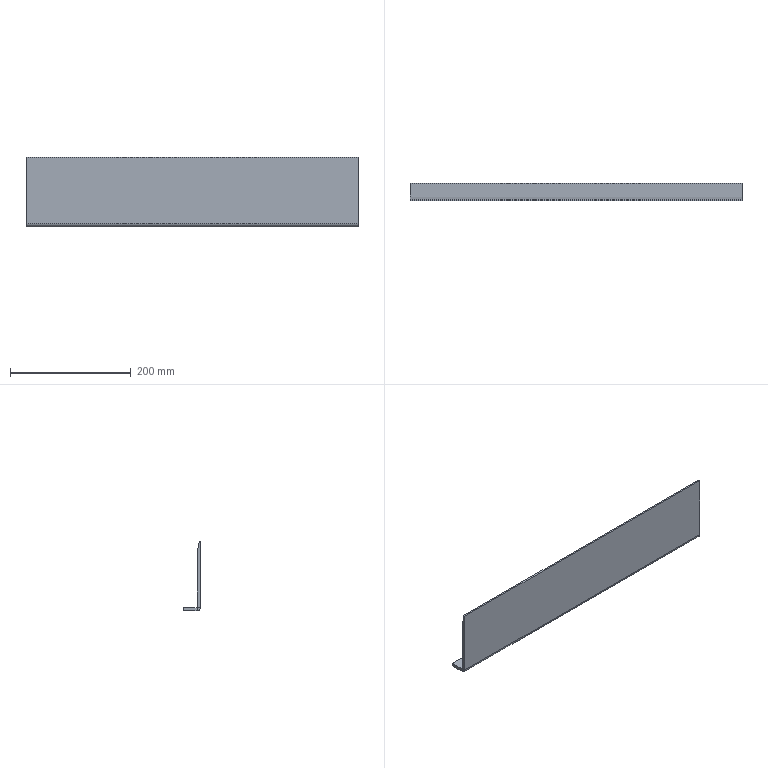Component | SolidWorks | PusherTray-1 | 1 solid | 15 faces | box 550 x 29 x 115.5 mm | volume 402219 mm3 | plane 13 | cylinder 2 | commonest cylinder face diameters 1 x1 12 x1
STEP:
#1=COLOUR_RGB('',0.7922,0.8196,0.9333);
#2=FILL_AREA_STYLE_COLOUR('',#1);
#3=FILL_AREA_STYLE('',(#2));
#4=SURFACE_STYLE_FILL_AREA(#3);
#5=SURFACE_SIDE_STYLE('',(#4));
#6=SURFACE_STYLE_USAGE(.BOTH.,#5);
#7=PRESENTATION_STYLE_ASSIGNMENT((#6));
#8=CARTESIAN_POINT('',(0.9843,24.724,0.8858));
#9=VERTEX_POINT('',#8);
#10=CARTESIAN_POINT('',(0.9843,24.508,0.8858));
#11=VERTEX_POINT('',#10);
#12=CARTESIAN_POINT('',(0.9843,24.724,0.8858));
#13=DIRECTION('',(0.,-1.,-0.));
#14=VECTOR('',#13,39.37);
#15=LINE('',#12,#14);
#16=EDGE_CURVE('',#9,#11,#15,.T.);
#17=ORIENTED_EDGE('',*,*,#16,.F.);
#18=CARTESIAN_POINT('',(0.9843,24.744,0.8661));
#19=VERTEX_POINT('',#18);
#20=CARTESIAN_POINT('',(0.9843,24.744,0.8858));
#21=DIRECTION('',(-1.,-0.,0.));
#22=DIRECTION('',(0.,0.,-1.));
#23=AXIS2_PLACEMENT_3D('',#20,#21,#22);
#24=CIRCLE('',#23,0.01969);
#25=EDGE_CURVE('',#19,#9,#24,.T.);
#26=ORIENTED_EDGE('',*,*,#25,.F.);
#27=CARTESIAN_POINT('',(0.9843,24.744,0.6496));
#28=VERTEX_POINT('',#27);
#29=CARTESIAN_POINT('',(0.9843,24.744,0.6496));
#30=DIRECTION('',(0.,-0.,1.));
#31=VECTOR('',#30,39.37);
#32=LINE('',#29,#31);
#33=EDGE_CURVE('',#28,#19,#32,.T.);
#34=ORIENTED_EDGE('',*,*,#33,.F.);
#35=CARTESIAN_POINT('',(0.9843,24.744,0.8858));
#36=DIRECTION('',(-1.,-0.,0.));
#37=DIRECTION('',(0.,0.,1.));
#38=AXIS2_PLACEMENT_3D('',#35,#36,#37);
#39=CIRCLE('',#38,0.2362);
#40=EDGE_CURVE('',#28,#11,#39,.T.);
#41=ORIENTED_EDGE('',*,*,#40,.T.);
#42=EDGE_LOOP('',(#17,#26,#34,#41));
#43=FACE_OUTER_BOUND('',#42,.T.);
#44=CARTESIAN_POINT('',(0.9843,24.724,0.8858));
#45=DIRECTION('',(-1.,-0.,0.));
#46=DIRECTION('',(0.,-0.,1.));
#47=AXIS2_PLACEMENT_3D('',#44,#45,#46);
#48=PLANE('',#47);
#49=ADVANCED_FACE('',(#43),#48,.T.);
#50=CARTESIAN_POINT('',(0.9843,24.606,5.197));
#51=VERTEX_POINT('',#50);
#52=CARTESIAN_POINT('',(0.9843,24.508,5.197));
#53=VERTEX_POINT('',#52);
#54=CARTESIAN_POINT('',(0.9843,24.724,5.197));
#55=DIRECTION('',(0.,-1.,-0.));
#56=VECTOR('',#55,39.37);
#57=LINE('',#54,#56);
#58=EDGE_CURVE('',#51,#53,#57,.T.);
#59=ORIENTED_EDGE('',*,*,#58,.F.);
#60=CARTESIAN_POINT('',(0.9843,24.724,4.527));
#61=VERTEX_POINT('',#60);
#62=CARTESIAN_POINT('',(0.9843,25.388,0.7632));
#63=DIRECTION('',(-0.,0.1736,-0.9848));
#64=VECTOR('',#63,39.37);
#65=LINE('',#62,#64);
#66=EDGE_CURVE('',#51,#61,#65,.T.);
#67=ORIENTED_EDGE('',*,*,#66,.T.);
#68=CARTESIAN_POINT('',(0.9843,24.724,0.8661));
#69=DIRECTION('',(0.,-0.,1.));
#70=VECTOR('',#69,39.37);
#71=LINE('',#68,#70);
#72=EDGE_CURVE('',#9,#61,#71,.T.);
#73=ORIENTED_EDGE('',*,*,#72,.F.);
#74=ORIENTED_EDGE('',*,*,#16,.T.);
#75=CARTESIAN_POINT('',(0.9843,24.508,0.8661));
#76=DIRECTION('',(0.,-0.,1.));
#77=VECTOR('',#76,39.37);
#78=LINE('',#75,#77);
#79=EDGE_CURVE('',#11,#53,#78,.T.);
#80=ORIENTED_EDGE('',*,*,#79,.T.);
#81=EDGE_LOOP('',(#59,#67,#73,#74,#80));
#82=FACE_OUTER_BOUND('',#81,.T.);
#83=CARTESIAN_POINT('',(0.9843,24.744,0.6496));
#84=DIRECTION('',(-1.,-0.,0.));
#85=DIRECTION('',(0.,-0.,1.));
#86=AXIS2_PLACEMENT_3D('',#83,#84,#85);
#87=PLANE('',#86);
#88=ADVANCED_FACE('',(#82),#87,.T.);
#89=CARTESIAN_POINT('',(22.638,24.744,0.8661));
#90=VERTEX_POINT('',#89);
#91=CARTESIAN_POINT('',(22.638,24.744,0.6496));
#92=VERTEX_POINT('',#91);
#93=CARTESIAN_POINT('',(22.638,24.744,0.8661));
#94=DIRECTION('',(-0.,0.,-1.));
#95=VECTOR('',#94,39.37);
#96=LINE('',#93,#95);
#97=EDGE_CURVE('',#90,#92,#96,.T.);
#98=ORIENTED_EDGE('',*,*,#97,.F.);
#99=CARTESIAN_POINT('',(22.638,24.724,0.8858));
#100=VERTEX_POINT('',#99);
#101=CARTESIAN_POINT('',(22.638,24.744,0.8858));
#102=DIRECTION('',(-1.,-0.,0.));
#103=DIRECTION('',(0.,0.,-1.));
#104=AXIS2_PLACEMENT_3D('',#101,#102,#103);
#105=CIRCLE('',#104,0.01969);
#106=EDGE_CURVE('',#90,#100,#105,.T.);
#107=ORIENTED_EDGE('',*,*,#106,.T.);
#108=CARTESIAN_POINT('',(22.638,24.508,0.8858));
#109=VERTEX_POINT('',#108);
#110=CARTESIAN_POINT('',(22.638,24.508,0.8858));
#111=DIRECTION('',(-0.,1.,0.));
#112=VECTOR('',#111,39.37);
#113=LINE('',#110,#112);
#114=EDGE_CURVE('',#109,#100,#113,.T.);
#115=ORIENTED_EDGE('',*,*,#114,.F.);
#116=CARTESIAN_POINT('',(22.638,24.744,0.8858));
#117=DIRECTION('',(-1.,-0.,0.));
#118=DIRECTION('',(0.,0.,1.));
#119=AXIS2_PLACEMENT_3D('',#116,#117,#118);
#120=CIRCLE('',#119,0.2362);
#121=EDGE_CURVE('',#92,#109,#120,.T.);
#122=ORIENTED_EDGE('',*,*,#121,.F.);
#123=EDGE_LOOP('',(#98,#107,#115,#122));
#124=FACE_OUTER_BOUND('',#123,.T.);
#125=CARTESIAN_POINT('',(22.638,24.744,0.8661));
#126=DIRECTION('',(1.,0.,-0.));
#127=DIRECTION('',(-0.,0.,-1.));
#128=AXIS2_PLACEMENT_3D('',#125,#126,#127);
#129=PLANE('',#128);
#130=ADVANCED_FACE('',(#124),#129,.T.);
#131=CARTESIAN_POINT('',(22.638,25.65,0.8661));
#132=VERTEX_POINT('',#131);
#133=CARTESIAN_POINT('',(22.638,24.724,0.8661));
#134=DIRECTION('',(0.,-1.,-0.));
#135=VECTOR('',#134,39.37);
#136=LINE('',#133,#135);
#137=EDGE_CURVE('',#132,#90,#136,.T.);
#138=ORIENTED_EDGE('',*,*,#137,.T.);
#139=ORIENTED_EDGE('',*,*,#97,.T.);
#140=CARTESIAN_POINT('',(22.638,25.65,0.6496));
#141=VERTEX_POINT('',#140);
#142=CARTESIAN_POINT('',(22.638,24.724,0.6496));
#143=DIRECTION('',(0.,-1.,-0.));
#144=VECTOR('',#143,39.37);
#145=LINE('',#142,#144);
#146=EDGE_CURVE('',#141,#92,#145,.T.);
#147=ORIENTED_EDGE('',*,*,#146,.F.);
#148=CARTESIAN_POINT('',(22.638,25.65,0.6496));
#149=DIRECTION('',(0.,-0.,1.));
#150=VECTOR('',#149,39.37);
#151=LINE('',#148,#150);
#152=EDGE_CURVE('',#141,#132,#151,.T.);
#153=ORIENTED_EDGE('',*,*,#152,.T.);
#154=EDGE_LOOP('',(#138,#139,#147,#153));
#155=FACE_OUTER_BOUND('',#154,.T.);
#156=CARTESIAN_POINT('',(22.638,24.508,0.8858));
#157=DIRECTION('',(1.,0.,-0.));
#158=DIRECTION('',(-0.,0.,-1.));
#159=AXIS2_PLACEMENT_3D('',#156,#157,#158);
#160=PLANE('',#159);
#161=ADVANCED_FACE('',(#155),#160,.T.);
#162=CARTESIAN_POINT('',(22.638,24.508,5.197));
#163=VERTEX_POINT('',#162);
#164=CARTESIAN_POINT('',(22.638,24.508,0.8661));
#165=DIRECTION('',(0.,-0.,1.));
#166=VECTOR('',#165,39.37);
#167=LINE('',#164,#166);
#168=EDGE_CURVE('',#109,#163,#167,.T.);
#169=ORIENTED_EDGE('',*,*,#168,.T.);
#170=CARTESIAN_POINT('',(0.9843,24.508,5.197));
#171=DIRECTION('',(1.,0.,-0.));
#172=VECTOR('',#171,39.37);
#173=LINE('',#170,#172);
#174=EDGE_CURVE('',#53,#163,#173,.T.);
#175=ORIENTED_EDGE('',*,*,#174,.F.);
#176=ORIENTED_EDGE('',*,*,#79,.F.);
#177=CARTESIAN_POINT('',(0.9843,24.508,0.8858));
#178=DIRECTION('',(1.,0.,-0.));
#179=VECTOR('',#178,39.37);
#180=LINE('',#177,#179);
#181=EDGE_CURVE('',#11,#109,#180,.T.);
#182=ORIENTED_EDGE('',*,*,#181,.T.);
#183=EDGE_LOOP('',(#169,#175,#176,#182));
#184=FACE_OUTER_BOUND('',#183,.T.);
#185=CARTESIAN_POINT('',(0.9843,24.508,0.8661));
#186=DIRECTION('',(-0.,1.,0.));
#187=DIRECTION('',(-1.,-0.,0.));
#188=AXIS2_PLACEMENT_3D('',#185,#186,#187);
#189=PLANE('',#188);
#190=ADVANCED_FACE('',(#184),#189,.F.);
#191=CARTESIAN_POINT('',(22.638,24.606,5.197));
#192=VERTEX_POINT('',#191);
#193=CARTESIAN_POINT('',(22.638,24.724,5.197));
#194=DIRECTION('',(0.,-1.,-0.));
#195=VECTOR('',#194,39.37);
#196=LINE('',#193,#195);
#197=EDGE_CURVE('',#192,#163,#196,.T.);
#198=ORIENTED_EDGE('',*,*,#197,.F.);
#199=CARTESIAN_POINT('',(0.9843,24.606,5.197));
#200=DIRECTION('',(-1.,-0.,0.));
#201=VECTOR('',#200,39.37);
#202=LINE('',#199,#201);
#203=EDGE_CURVE('',#192,#51,#202,.T.);
#204=ORIENTED_EDGE('',*,*,#203,.T.);
#205=ORIENTED_EDGE('',*,*,#58,.T.);
#206=ORIENTED_EDGE('',*,*,#174,.T.);
#207=EDGE_LOOP('',(#198,#204,#205,#206));
#208=FACE_OUTER_BOUND('',#207,.T.);
#209=CARTESIAN_POINT('',(0.9843,24.724,5.197));
#210=DIRECTION('',(0.,-0.,1.));
#211=DIRECTION('',(1.,0.,-0.));
#212=AXIS2_PLACEMENT_3D('',#209,#210,#211);
#213=PLANE('',#212);
#214=ADVANCED_FACE('',(#208),#213,.T.);
#215=ORIENTED_EDGE('',*,*,#72,.T.);
#216=CARTESIAN_POINT('',(22.638,24.724,4.527));
#217=VERTEX_POINT('',#216);
#218=CARTESIAN_POINT('',(0.9843,24.724,4.527));
#219=DIRECTION('',(1.,0.,-0.));
#220=VECTOR('',#219,39.37);
#221=LINE('',#218,#220);
#222=EDGE_CURVE('',#61,#217,#221,.T.);
#223=ORIENTED_EDGE('',*,*,#222,.T.);
#224=CARTESIAN_POINT('',(22.638,24.724,0.8661));
#225=DIRECTION('',(0.,-0.,1.));
#226=VECTOR('',#225,39.37);
#227=LINE('',#224,#226);
#228=EDGE_CURVE('',#100,#217,#227,.T.);
#229=ORIENTED_EDGE('',*,*,#228,.F.);
#230=CARTESIAN_POINT('',(0.9843,24.724,0.8858));
#231=DIRECTION('',(1.,0.,-0.));
#232=VECTOR('',#231,39.37);
#233=LINE('',#230,#232);
#234=EDGE_CURVE('',#9,#100,#233,.T.);
#235=ORIENTED_EDGE('',*,*,#234,.F.);
#236=EDGE_LOOP('',(#215,#223,#229,#235));
#237=FACE_OUTER_BOUND('',#236,.T.);
#238=CARTESIAN_POINT('',(0.9843,24.724,0.8661));
#239=DIRECTION('',(-0.,1.,0.));
#240=DIRECTION('',(-1.,-0.,0.));
#241=AXIS2_PLACEMENT_3D('',#238,#239,#240);
#242=PLANE('',#241);
#243=ADVANCED_FACE('',(#237),#242,.T.);
#244=ORIENTED_EDGE('',*,*,#106,.F.);
#245=CARTESIAN_POINT('',(0.9843,24.744,0.8661));
#246=DIRECTION('',(1.,0.,-0.));
#247=VECTOR('',#246,39.37);
#248=LINE('',#245,#247);
#249=EDGE_CURVE('',#19,#90,#248,.T.);
#250=ORIENTED_EDGE('',*,*,#249,.F.);
#251=ORIENTED_EDGE('',*,*,#25,.T.);
#252=ORIENTED_EDGE('',*,*,#234,.T.);
#253=EDGE_LOOP('',(#244,#250,#251,#252));
#254=FACE_OUTER_BOUND('',#253,.T.);
#255=CARTESIAN_POINT('',(0.9843,24.744,0.8858));
#256=DIRECTION('',(1.,0.,-0.));
#257=DIRECTION('',(0.,0.,-1.));
#258=AXIS2_PLACEMENT_3D('',#255,#256,#257);
#259=CYLINDRICAL_SURFACE('',#258,0.01969);
#260=ADVANCED_FACE('',(#254),#259,.F.);
#261=ORIENTED_EDGE('',*,*,#137,.F.);
#262=CARTESIAN_POINT('',(0.9843,25.65,0.8661));
#263=VERTEX_POINT('',#262);
#264=CARTESIAN_POINT('',(0.9843,25.65,0.8661));
#265=DIRECTION('',(1.,0.,-0.));
#266=VECTOR('',#265,39.37);
#267=LINE('',#264,#266);
#268=EDGE_CURVE('',#263,#132,#267,.T.);
#269=ORIENTED_EDGE('',*,*,#268,.F.);
#270=CARTESIAN_POINT('',(0.9843,24.724,0.8661));
#271=DIRECTION('',(0.,-1.,-0.));
#272=VECTOR('',#271,39.37);
#273=LINE('',#270,#272);
#274=EDGE_CURVE('',#263,#19,#273,.T.);
#275=ORIENTED_EDGE('',*,*,#274,.T.);
#276=ORIENTED_EDGE('',*,*,#249,.T.);
#277=EDGE_LOOP('',(#261,#269,#275,#276));
#278=FACE_OUTER_BOUND('',#277,.T.);
#279=CARTESIAN_POINT('',(0.9843,24.724,0.8661));
#280=DIRECTION('',(0.,-0.,1.));
#281=DIRECTION('',(1.,0.,-0.));
#282=AXIS2_PLACEMENT_3D('',#279,#280,#281);
#283=PLANE('',#282);
#284=ADVANCED_FACE('',(#278),#283,.T.);
#285=ORIENTED_EDGE('',*,*,#152,.F.);
#286=CARTESIAN_POINT('',(0.9843,25.65,0.6496));
#287=VERTEX_POINT('',#286);
#288=CARTESIAN_POINT('',(0.9843,25.65,0.6496));
#289=DIRECTION('',(1.,0.,-0.));
#290=VECTOR('',#289,39.37);
#291=LINE('',#288,#290);
#292=EDGE_CURVE('',#287,#141,#291,.T.);
#293=ORIENTED_EDGE('',*,*,#292,.F.);
#294=CARTESIAN_POINT('',(0.9843,25.65,0.6496));
#295=DIRECTION('',(0.,-0.,1.));
#296=VECTOR('',#295,39.37);
#297=LINE('',#294,#296);
#298=EDGE_CURVE('',#287,#263,#297,.T.);
#299=ORIENTED_EDGE('',*,*,#298,.T.);
#300=ORIENTED_EDGE('',*,*,#268,.T.);
#301=EDGE_LOOP('',(#285,#293,#299,#300));
#302=FACE_OUTER_BOUND('',#301,.T.);
#303=CARTESIAN_POINT('',(0.9843,25.65,0.6496));
#304=DIRECTION('',(-0.,1.,0.));
#305=DIRECTION('',(-1.,-0.,0.));
#306=AXIS2_PLACEMENT_3D('',#303,#304,#305);
#307=PLANE('',#306);
#308=ADVANCED_FACE('',(#302),#307,.T.);
#309=ORIENTED_EDGE('',*,*,#146,.T.);
#310=CARTESIAN_POINT('',(0.9843,24.744,0.6496));
#311=DIRECTION('',(1.,0.,-0.));
#312=VECTOR('',#311,39.37);
#313=LINE('',#310,#312);
#314=EDGE_CURVE('',#28,#92,#313,.T.);
#315=ORIENTED_EDGE('',*,*,#314,.F.);
#316=CARTESIAN_POINT('',(0.9843,24.724,0.6496));
#317=DIRECTION('',(0.,-1.,-0.));
#318=VECTOR('',#317,39.37);
#319=LINE('',#316,#318);
#320=EDGE_CURVE('',#287,#28,#319,.T.);
#321=ORIENTED_EDGE('',*,*,#320,.F.);
#322=ORIENTED_EDGE('',*,*,#292,.T.);
#323=EDGE_LOOP('',(#309,#315,#321,#322));
#324=FACE_OUTER_BOUND('',#323,.T.);
#325=CARTESIAN_POINT('',(0.9843,24.724,0.6496));
#326=DIRECTION('',(0.,-0.,1.));
#327=DIRECTION('',(1.,0.,-0.));
#328=AXIS2_PLACEMENT_3D('',#325,#326,#327);
#329=PLANE('',#328);
#330=ADVANCED_FACE('',(#324),#329,.F.);
#331=ORIENTED_EDGE('',*,*,#121,.T.);
#332=ORIENTED_EDGE('',*,*,#181,.F.);
#333=ORIENTED_EDGE('',*,*,#40,.F.);
#334=ORIENTED_EDGE('',*,*,#314,.T.);
#335=EDGE_LOOP('',(#331,#332,#333,#334));
#336=FACE_OUTER_BOUND('',#335,.T.);
#337=CARTESIAN_POINT('',(0.9843,24.744,0.8858));
#338=DIRECTION('',(1.,0.,-0.));
#339=DIRECTION('',(0.,0.,-1.));
#340=AXIS2_PLACEMENT_3D('',#337,#338,#339);
#341=CYLINDRICAL_SURFACE('',#340,0.2362);
#342=ADVANCED_FACE('',(#336),#341,.T.);
#343=ORIENTED_EDGE('',*,*,#320,.T.);
#344=ORIENTED_EDGE('',*,*,#33,.T.);
#345=ORIENTED_EDGE('',*,*,#274,.F.);
#346=ORIENTED_EDGE('',*,*,#298,.F.);
#347=EDGE_LOOP('',(#343,#344,#345,#346));
#348=FACE_OUTER_BOUND('',#347,.T.);
#349=CARTESIAN_POINT('',(0.9843,24.744,0.8858));
#350=DIRECTION('',(1.,0.,-0.));
#351=DIRECTION('',(-0.,0.,-1.));
#352=AXIS2_PLACEMENT_3D('',#349,#350,#351);
#353=PLANE('',#352);
#354=ADVANCED_FACE('',(#348),#353,.F.);
#355=ORIENTED_EDGE('',*,*,#228,.T.);
#356=CARTESIAN_POINT('',(22.638,25.348,0.9923));
#357=DIRECTION('',(0.,-0.1736,0.9848));
#358=VECTOR('',#357,39.37);
#359=LINE('',#356,#358);
#360=EDGE_CURVE('',#217,#192,#359,.T.);
#361=ORIENTED_EDGE('',*,*,#360,.T.);
#362=ORIENTED_EDGE('',*,*,#197,.T.);
#363=ORIENTED_EDGE('',*,*,#168,.F.);
#364=ORIENTED_EDGE('',*,*,#114,.T.);
#365=EDGE_LOOP('',(#355,#361,#362,#363,#364));
#366=FACE_OUTER_BOUND('',#365,.T.);
#367=CARTESIAN_POINT('',(22.638,24.744,0.8858));
#368=DIRECTION('',(1.,0.,-0.));
#369=DIRECTION('',(-0.,0.,-1.));
#370=AXIS2_PLACEMENT_3D('',#367,#368,#369);
#371=PLANE('',#370);
#372=ADVANCED_FACE('',(#366),#371,.T.);
#373=ORIENTED_EDGE('',*,*,#66,.F.);
#374=ORIENTED_EDGE('',*,*,#203,.F.);
#375=ORIENTED_EDGE('',*,*,#360,.F.);
#376=ORIENTED_EDGE('',*,*,#222,.F.);
#377=EDGE_LOOP('',(#373,#374,#375,#376));
#378=FACE_OUTER_BOUND('',#377,.T.);
#379=CARTESIAN_POINT('',(0.9843,24.724,4.527));
#380=DIRECTION('',(0.,-0.9848,-0.1736));
#381=DIRECTION('',(1.,0.,-0.));
#382=AXIS2_PLACEMENT_3D('',#379,#380,#381);
#383=PLANE('',#382);
#384=ADVANCED_FACE('',(#378),#383,.F.);
#385=CLOSED_SHELL('',(#49,#88,#130,#161,#190,#214,#243,#260,#284,#308,#330,#342,#354,#372,#384));
#386=MANIFOLD_SOLID_BREP('',#385);
#387=STYLED_ITEM('',(#7),#386);
#388=PRESENTATION_LAYER_ASSIGNMENT('','',(#387));
#389=CARTESIAN_POINT('',(0.,0.,0.));
#390=DIRECTION('',(0.,0.,1.));
#391=DIRECTION('',(1.,0.,0.));
#392=AXIS2_PLACEMENT_3D('',#389,#390,#391);
#393=(LENGTH_UNIT()NAMED_UNIT(*)SI_UNIT($,.METRE.));
#394=LENGTH_MEASURE_WITH_UNIT(LENGTH_MEASURE(0.0254),#393);
#395=DIMENSIONAL_EXPONENTS(1.,0.,0.,0.,0.,0.,0.);
#396=(CONVERSION_BASED_UNIT('',#394)LENGTH_UNIT()NAMED_UNIT(#395));
#397=UNCERTAINTY_MEASURE_WITH_UNIT(LENGTH_MEASURE(0.00001),#396,'','');
#398=(NAMED_UNIT(*)PLANE_ANGLE_UNIT()SI_UNIT($,.RADIAN.));
#399=(NAMED_UNIT(*)SI_UNIT($,.STERADIAN.)SOLID_ANGLE_UNIT());
#400=(GEOMETRIC_REPRESENTATION_CONTEXT(3)GLOBAL_UNCERTAINTY_ASSIGNED_CONTEXT((#397))GLOBAL_UNIT_ASSIGNED_CONTEXT((#396,#398,#399))REPRESENTATION_CONTEXT('',''));
#401=ADVANCED_BREP_SHAPE_REPRESENTATION('',(#386,#392),#400);
#402=(LENGTH_UNIT()NAMED_UNIT(*)SI_UNIT($,.METRE.));
#403=LENGTH_MEASURE_WITH_UNIT(LENGTH_MEASURE(0.0254),#402);
#404=DIMENSIONAL_EXPONENTS(1.,0.,0.,0.,0.,0.,0.);
#405=(CONVERSION_BASED_UNIT('',#403)LENGTH_UNIT()NAMED_UNIT(#404));
#406=UNCERTAINTY_MEASURE_WITH_UNIT(LENGTH_MEASURE(0.00001),#405,'','');
#407=(NAMED_UNIT(*)PLANE_ANGLE_UNIT()SI_UNIT($,.RADIAN.));
#408=(NAMED_UNIT(*)SI_UNIT($,.STERADIAN.)SOLID_ANGLE_UNIT());
#409=(GEOMETRIC_REPRESENTATION_CONTEXT(3)GLOBAL_UNCERTAINTY_ASSIGNED_CONTEXT((#406))GLOBAL_UNIT_ASSIGNED_CONTEXT((#405,#407,#408))REPRESENTATION_CONTEXT('',''));
#410=MECHANICAL_DESIGN_GEOMETRIC_PRESENTATION_REPRESENTATION('',(#387),#409);